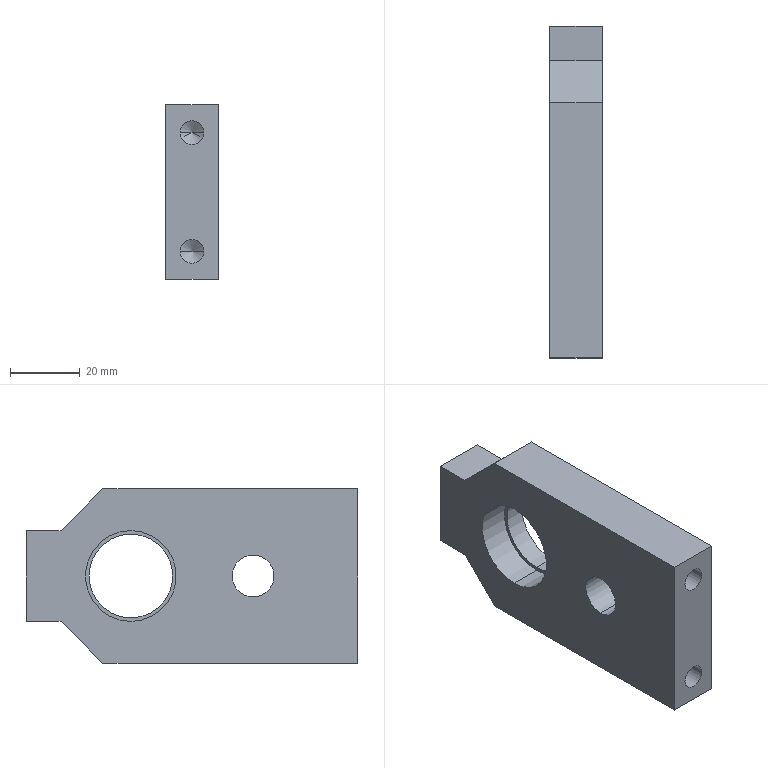Component | SolidWorks | BracketTwo-2 | 1 solid | 25 faces | box 15 x 95 x 50 mm | volume 55307 mm3 | plane 11 | cylinder 10 | cone 4 | commonest cylinder face diameters 6.8 x4 24 x2 26 x2 12 x2
build123d program:
from build123d import *

# Parameters (mm, degrees)
SKETCH1_R             = 6
BOSS_EXTRUDE1_DEPTH   = 15
SKETCH2_R             = 13
CUT_EXTRUDE1_DEPTH    = 9
SKETCH3_R             = 12
CUT_EXTRUDE2_DEPTH    = 6
M8_TAPPED_HOLE1_D     = 6.8
M8_TAPPED_HOLE1_DEPTH = 13
M8_TAPPED_HOLE1_TIP   = 2.043
SKETCH7_W             = 26
SKETCH7_H             = 15
BOSS_EXTRUDE2_DEPTH   = 10


with BuildPart() as part:
    # Sketch1 → Boss-Extrude1 (new body)
    with BuildSketch(Plane.XY):
        Polygon((-25, 30.5), (-13, 42.5), (13, 42.5), (25, 30.5), (25, -42.5), (-25, -42.5), align=None)
        with Locations((0, -12.5)):
            Circle(SKETCH1_R, mode=Mode.SUBTRACT)
    extrude(amount=BOSS_EXTRUDE1_DEPTH)

    # Sketch2 → Cut-Extrude1 (cut)
    with BuildSketch(Plane.XY.offset(15)):
        with Locations((0, 22.5)):
            Circle(SKETCH2_R)
    extrude(amount=-CUT_EXTRUDE1_DEPTH, mode=Mode.SUBTRACT)

    # Sketch3 → Cut-Extrude2 (cut)
    with BuildSketch(Plane.XY.offset(6)):
        with Locations((0, 22.5)):
            Circle(SKETCH3_R)
    extrude(amount=-CUT_EXTRUDE2_DEPTH, mode=Mode.SUBTRACT)

    # M8 Tapped Hole1
    with Locations(Plane(origin=(0, -42.5, 0), x_dir=(-1, 0, 0), z_dir=(0, -1, 0))):
        with Locations((17, -7.5), (-17, -7.5)):
            Hole(M8_TAPPED_HOLE1_D / 2, depth=M8_TAPPED_HOLE1_DEPTH)
            with Locations((0, 0, -(M8_TAPPED_HOLE1_DEPTH + M8_TAPPED_HOLE1_TIP / 2))):  # 118° drill point
                Cone(0, M8_TAPPED_HOLE1_D / 2, M8_TAPPED_HOLE1_TIP, mode=Mode.SUBTRACT)

    # Sketch7 → Boss-Extrude2 (add)
    with BuildSketch(Plane(origin=(0, 42.5, 0), x_dir=(1, 0, 0), z_dir=(0, 1, 0))):
        with Locations((0, -7.5)):
            Rectangle(SKETCH7_W, SKETCH7_H)
    extrude(amount=BOSS_EXTRUDE2_DEPTH)


solid = part.part

# Placed as in the assembly
solid = solid.moved(Location((195.546, 54.5, 438.671), (0, -90, 0)))
STEP:
#1=COLOUR_RGB('',0.7922,0.8196,0.9333);
#2=FILL_AREA_STYLE_COLOUR('',#1);
#3=FILL_AREA_STYLE('',(#2));
#4=SURFACE_STYLE_FILL_AREA(#3);
#5=SURFACE_SIDE_STYLE('',(#4));
#6=SURFACE_STYLE_USAGE(.BOTH.,#5);
#7=PRESENTATION_STYLE_ASSIGNMENT((#6));
#8=CARTESIAN_POINT('',(7.27,0.9843,16.601));
#9=VERTEX_POINT('',#8);
#10=CARTESIAN_POINT('',(7.537,0.9843,16.601));
#11=VERTEX_POINT('',#10);
#12=CARTESIAN_POINT('',(7.403,0.9843,16.601));
#13=DIRECTION('',(0.,-1.,0.));
#14=DIRECTION('',(1.,0.,-0.));
#15=AXIS2_PLACEMENT_3D('',#12,#13,#14);
#16=CIRCLE('',#15,0.1339);
#17=EDGE_CURVE('',#9,#11,#16,.T.);
#18=ORIENTED_EDGE('',*,*,#17,.F.);
#19=CARTESIAN_POINT('',(7.27,0.4724,16.601));
#20=VERTEX_POINT('',#19);
#21=CARTESIAN_POINT('',(7.27,0.4724,16.601));
#22=DIRECTION('',(0.,-1.,0.));
#23=VECTOR('',#22,39.37);
#24=LINE('',#21,#23);
#25=EDGE_CURVE('',#9,#20,#24,.T.);
#26=ORIENTED_EDGE('',*,*,#25,.T.);
#27=CARTESIAN_POINT('',(7.537,0.4724,16.601));
#28=VERTEX_POINT('',#27);
#29=CARTESIAN_POINT('',(7.403,0.4724,16.601));
#30=DIRECTION('',(0.,-1.,0.));
#31=DIRECTION('',(1.,0.,-0.));
#32=AXIS2_PLACEMENT_3D('',#29,#30,#31);
#33=CIRCLE('',#32,0.1339);
#34=EDGE_CURVE('',#20,#28,#33,.T.);
#35=ORIENTED_EDGE('',*,*,#34,.T.);
#36=CARTESIAN_POINT('',(7.537,0.4724,16.601));
#37=DIRECTION('',(0.,-1.,0.));
#38=VECTOR('',#37,39.37);
#39=LINE('',#36,#38);
#40=EDGE_CURVE('',#11,#28,#39,.T.);
#41=ORIENTED_EDGE('',*,*,#40,.F.);
#42=EDGE_LOOP('',(#18,#26,#35,#41));
#43=FACE_OUTER_BOUND('',#42,.T.);
#44=CARTESIAN_POINT('',(7.403,0.4724,16.601));
#45=DIRECTION('',(0.,-1.,0.));
#46=DIRECTION('',(1.,0.,-0.));
#47=AXIS2_PLACEMENT_3D('',#44,#45,#46);
#48=CYLINDRICAL_SURFACE('',#47,0.1339);
#49=ADVANCED_FACE('',(#43),#48,.F.);
#50=CARTESIAN_POINT('',(7.403,1.065,16.601));
#51=VERTEX_POINT('',#50);
#52=CARTESIAN_POINT('',(7.537,0.9843,16.601));
#53=DIRECTION('',(0.8572,-0.515,-0.));
#54=VECTOR('',#53,39.37);
#55=LINE('',#52,#54);
#56=EDGE_CURVE('',#51,#11,#55,.T.);
#57=ORIENTED_EDGE('',*,*,#56,.F.);
#58=CARTESIAN_POINT('',(7.27,0.9843,16.601));
#59=DIRECTION('',(-0.8572,-0.515,0.));
#60=VECTOR('',#59,39.37);
#61=LINE('',#58,#60);
#62=EDGE_CURVE('',#51,#9,#61,.T.);
#63=ORIENTED_EDGE('',*,*,#62,.T.);
#64=ORIENTED_EDGE('',*,*,#17,.T.);
#65=EDGE_LOOP('',(#57,#63,#64));
#66=FACE_OUTER_BOUND('',#65,.T.);
#67=CARTESIAN_POINT('',(7.403,0.9843,16.601));
#68=DIRECTION('',(0.,-1.,0.));
#69=DIRECTION('',(1.,0.,-0.));
#70=AXIS2_PLACEMENT_3D('',#67,#68,#69);
#71=CONICAL_SURFACE('',#70,0.1339,1.03);
#72=ADVANCED_FACE('',(#66),#71,.F.);
#73=CARTESIAN_POINT('',(7.27,0.9843,17.94));
#74=VERTEX_POINT('',#73);
#75=CARTESIAN_POINT('',(7.537,0.9843,17.94));
#76=VERTEX_POINT('',#75);
#77=CARTESIAN_POINT('',(7.403,0.9843,17.94));
#78=DIRECTION('',(0.,-1.,0.));
#79=DIRECTION('',(1.,0.,-0.));
#80=AXIS2_PLACEMENT_3D('',#77,#78,#79);
#81=CIRCLE('',#80,0.1339);
#82=EDGE_CURVE('',#74,#76,#81,.T.);
#83=ORIENTED_EDGE('',*,*,#82,.F.);
#84=CARTESIAN_POINT('',(7.27,0.4724,17.94));
#85=VERTEX_POINT('',#84);
#86=CARTESIAN_POINT('',(7.27,0.4724,17.94));
#87=DIRECTION('',(0.,-1.,0.));
#88=VECTOR('',#87,39.37);
#89=LINE('',#86,#88);
#90=EDGE_CURVE('',#74,#85,#89,.T.);
#91=ORIENTED_EDGE('',*,*,#90,.T.);
#92=CARTESIAN_POINT('',(7.537,0.4724,17.94));
#93=VERTEX_POINT('',#92);
#94=CARTESIAN_POINT('',(7.403,0.4724,17.94));
#95=DIRECTION('',(0.,-1.,0.));
#96=DIRECTION('',(1.,0.,-0.));
#97=AXIS2_PLACEMENT_3D('',#94,#95,#96);
#98=CIRCLE('',#97,0.1339);
#99=EDGE_CURVE('',#85,#93,#98,.T.);
#100=ORIENTED_EDGE('',*,*,#99,.T.);
#101=CARTESIAN_POINT('',(7.537,0.4724,17.94));
#102=DIRECTION('',(0.,-1.,0.));
#103=VECTOR('',#102,39.37);
#104=LINE('',#101,#103);
#105=EDGE_CURVE('',#76,#93,#104,.T.);
#106=ORIENTED_EDGE('',*,*,#105,.F.);
#107=EDGE_LOOP('',(#83,#91,#100,#106));
#108=FACE_OUTER_BOUND('',#107,.T.);
#109=CARTESIAN_POINT('',(7.403,0.4724,17.94));
#110=DIRECTION('',(0.,-1.,0.));
#111=DIRECTION('',(1.,0.,-0.));
#112=AXIS2_PLACEMENT_3D('',#109,#110,#111);
#113=CYLINDRICAL_SURFACE('',#112,0.1339);
#114=ADVANCED_FACE('',(#108),#113,.F.);
#115=CARTESIAN_POINT('',(7.403,1.065,17.94));
#116=VERTEX_POINT('',#115);
#117=CARTESIAN_POINT('',(7.537,0.9843,17.94));
#118=DIRECTION('',(0.8572,-0.515,-0.));
#119=VECTOR('',#118,39.37);
#120=LINE('',#117,#119);
#121=EDGE_CURVE('',#116,#76,#120,.T.);
#122=ORIENTED_EDGE('',*,*,#121,.F.);
#123=CARTESIAN_POINT('',(7.27,0.9843,17.94));
#124=DIRECTION('',(-0.8572,-0.515,0.));
#125=VECTOR('',#124,39.37);
#126=LINE('',#123,#125);
#127=EDGE_CURVE('',#116,#74,#126,.T.);
#128=ORIENTED_EDGE('',*,*,#127,.T.);
#129=ORIENTED_EDGE('',*,*,#82,.T.);
#130=EDGE_LOOP('',(#122,#128,#129));
#131=FACE_OUTER_BOUND('',#130,.T.);
#132=CARTESIAN_POINT('',(7.403,0.9843,17.94));
#133=DIRECTION('',(0.,-1.,0.));
#134=DIRECTION('',(1.,0.,-0.));
#135=AXIS2_PLACEMENT_3D('',#132,#133,#134);
#136=CONICAL_SURFACE('',#135,0.1339,1.03);
#137=ADVANCED_FACE('',(#131),#136,.F.);
#138=CARTESIAN_POINT('',(7.699,3.031,17.743));
#139=VERTEX_POINT('',#138);
#140=CARTESIAN_POINT('',(7.699,3.031,16.798));
#141=VERTEX_POINT('',#140);
#142=CARTESIAN_POINT('',(7.699,3.031,17.271));
#143=DIRECTION('',(1.,0.,-0.));
#144=DIRECTION('',(0.,0.,1.));
#145=AXIS2_PLACEMENT_3D('',#142,#143,#144);
#146=CIRCLE('',#145,0.4724);
#147=EDGE_CURVE('',#139,#141,#146,.T.);
#148=ORIENTED_EDGE('',*,*,#147,.T.);
#149=CARTESIAN_POINT('',(7.462,3.031,16.798));
#150=VERTEX_POINT('',#149);
#151=CARTESIAN_POINT('',(9.035,3.031,16.798));
#152=DIRECTION('',(-1.,-0.,0.));
#153=VECTOR('',#152,39.37);
#154=LINE('',#151,#153);
#155=EDGE_CURVE('',#141,#150,#154,.T.);
#156=ORIENTED_EDGE('',*,*,#155,.T.);
#157=CARTESIAN_POINT('',(7.462,3.031,17.743));
#158=VERTEX_POINT('',#157);
#159=CARTESIAN_POINT('',(7.462,3.031,17.271));
#160=DIRECTION('',(-1.,-0.,0.));
#161=DIRECTION('',(0.,0.,1.));
#162=AXIS2_PLACEMENT_3D('',#159,#160,#161);
#163=CIRCLE('',#162,0.4724);
#164=EDGE_CURVE('',#150,#158,#163,.T.);
#165=ORIENTED_EDGE('',*,*,#164,.T.);
#166=CARTESIAN_POINT('',(9.035,3.031,17.743));
#167=DIRECTION('',(-1.,-0.,0.));
#168=VECTOR('',#167,39.37);
#169=LINE('',#166,#168);
#170=EDGE_CURVE('',#139,#158,#169,.T.);
#171=ORIENTED_EDGE('',*,*,#170,.F.);
#172=EDGE_LOOP('',(#148,#156,#165,#171));
#173=FACE_OUTER_BOUND('',#172,.T.);
#174=CARTESIAN_POINT('',(9.035,3.031,17.271));
#175=DIRECTION('',(-1.,-0.,0.));
#176=DIRECTION('',(0.,0.,1.));
#177=AXIS2_PLACEMENT_3D('',#174,#175,#176);
#178=CYLINDRICAL_SURFACE('',#177,0.4724);
#179=ADVANCED_FACE('',(#173),#178,.F.);
#180=CARTESIAN_POINT('',(7.462,3.031,16.759));
#181=VERTEX_POINT('',#180);
#182=CARTESIAN_POINT('',(7.462,3.031,17.782));
#183=VERTEX_POINT('',#182);
#184=CARTESIAN_POINT('',(7.462,3.031,17.271));
#185=DIRECTION('',(-1.,-0.,0.));
#186=DIRECTION('',(0.,0.,1.));
#187=AXIS2_PLACEMENT_3D('',#184,#185,#186);
#188=CIRCLE('',#187,0.5118);
#189=EDGE_CURVE('',#181,#183,#188,.T.);
#190=ORIENTED_EDGE('',*,*,#189,.F.);
#191=CARTESIAN_POINT('',(7.108,3.031,16.759));
#192=VERTEX_POINT('',#191);
#193=CARTESIAN_POINT('',(7.462,3.031,16.759));
#194=DIRECTION('',(-1.,-0.,0.));
#195=VECTOR('',#194,39.37);
#196=LINE('',#193,#195);
#197=EDGE_CURVE('',#181,#192,#196,.T.);
#198=ORIENTED_EDGE('',*,*,#197,.T.);
#199=CARTESIAN_POINT('',(7.108,3.031,17.782));
#200=VERTEX_POINT('',#199);
#201=CARTESIAN_POINT('',(7.108,3.031,17.271));
#202=DIRECTION('',(-1.,-0.,0.));
#203=DIRECTION('',(0.,0.,1.));
#204=AXIS2_PLACEMENT_3D('',#201,#202,#203);
#205=CIRCLE('',#204,0.5118);
#206=EDGE_CURVE('',#192,#200,#205,.T.);
#207=ORIENTED_EDGE('',*,*,#206,.T.);
#208=CARTESIAN_POINT('',(7.462,3.031,17.782));
#209=DIRECTION('',(-1.,-0.,0.));
#210=VECTOR('',#209,39.37);
#211=LINE('',#208,#210);
#212=EDGE_CURVE('',#183,#200,#211,.T.);
#213=ORIENTED_EDGE('',*,*,#212,.F.);
#214=EDGE_LOOP('',(#190,#198,#207,#213));
#215=FACE_OUTER_BOUND('',#214,.T.);
#216=CARTESIAN_POINT('',(7.462,3.031,17.271));
#217=DIRECTION('',(-1.,-0.,0.));
#218=DIRECTION('',(0.,0.,1.));
#219=AXIS2_PLACEMENT_3D('',#216,#217,#218);
#220=CYLINDRICAL_SURFACE('',#219,0.5118);
#221=ADVANCED_FACE('',(#215),#220,.F.);
#222=CARTESIAN_POINT('',(7.108,1.654,17.034));
#223=VERTEX_POINT('',#222);
#224=CARTESIAN_POINT('',(7.108,1.654,17.507));
#225=VERTEX_POINT('',#224);
#226=CARTESIAN_POINT('',(7.108,1.654,17.271));
#227=DIRECTION('',(-1.,-0.,0.));
#228=DIRECTION('',(0.,0.,1.));
#229=AXIS2_PLACEMENT_3D('',#226,#227,#228);
#230=CIRCLE('',#229,0.2362);
#231=EDGE_CURVE('',#223,#225,#230,.T.);
#232=ORIENTED_EDGE('',*,*,#231,.T.);
#233=CARTESIAN_POINT('',(7.699,1.654,17.507));
#234=VERTEX_POINT('',#233);
#235=CARTESIAN_POINT('',(7.108,1.654,17.507));
#236=DIRECTION('',(1.,0.,-0.));
#237=VECTOR('',#236,39.37);
#238=LINE('',#235,#237);
#239=EDGE_CURVE('',#225,#234,#238,.T.);
#240=ORIENTED_EDGE('',*,*,#239,.T.);
#241=CARTESIAN_POINT('',(7.699,1.654,17.034));
#242=VERTEX_POINT('',#241);
#243=CARTESIAN_POINT('',(7.699,1.654,17.271));
#244=DIRECTION('',(-1.,-0.,0.));
#245=DIRECTION('',(0.,0.,1.));
#246=AXIS2_PLACEMENT_3D('',#243,#244,#245);
#247=CIRCLE('',#246,0.2362);
#248=EDGE_CURVE('',#242,#234,#247,.T.);
#249=ORIENTED_EDGE('',*,*,#248,.F.);
#250=CARTESIAN_POINT('',(7.108,1.654,17.034));
#251=DIRECTION('',(1.,0.,-0.));
#252=VECTOR('',#251,39.37);
#253=LINE('',#250,#252);
#254=EDGE_CURVE('',#223,#242,#253,.T.);
#255=ORIENTED_EDGE('',*,*,#254,.F.);
#256=EDGE_LOOP('',(#232,#240,#249,#255));
#257=FACE_OUTER_BOUND('',#256,.T.);
#258=CARTESIAN_POINT('',(7.108,1.654,17.271));
#259=DIRECTION('',(1.,0.,-0.));
#260=DIRECTION('',(-0.,0.,-1.));
#261=AXIS2_PLACEMENT_3D('',#258,#259,#260);
#262=CYLINDRICAL_SURFACE('',#261,0.2362);
#263=ADVANCED_FACE('',(#257),#262,.F.);
#264=CARTESIAN_POINT('',(7.108,3.031,17.271));
#265=DIRECTION('',(-1.,-0.,0.));
#266=DIRECTION('',(0.,0.,1.));
#267=AXIS2_PLACEMENT_3D('',#264,#265,#266);
#268=CIRCLE('',#267,0.5118);
#269=EDGE_CURVE('',#200,#192,#268,.T.);
#270=ORIENTED_EDGE('',*,*,#269,.F.);
#271=ORIENTED_EDGE('',*,*,#206,.F.);
#272=EDGE_LOOP('',(#270,#271));
#273=FACE_BOUND('',#272,.T.);
#274=CARTESIAN_POINT('',(7.108,0.4724,18.255));
#275=VERTEX_POINT('',#274);
#276=CARTESIAN_POINT('',(7.108,3.346,18.255));
#277=VERTEX_POINT('',#276);
#278=CARTESIAN_POINT('',(7.108,3.346,18.255));
#279=DIRECTION('',(-0.,1.,-0.));
#280=VECTOR('',#279,39.37);
#281=LINE('',#278,#280);
#282=EDGE_CURVE('',#275,#277,#281,.T.);
#283=ORIENTED_EDGE('',*,*,#282,.T.);
#284=CARTESIAN_POINT('',(7.108,3.819,17.782));
#285=VERTEX_POINT('',#284);
#286=CARTESIAN_POINT('',(7.108,3.819,17.782));
#287=DIRECTION('',(-0.,0.7071,-0.7071));
#288=VECTOR('',#287,39.37);
#289=LINE('',#286,#288);
#290=EDGE_CURVE('',#277,#285,#289,.T.);
#291=ORIENTED_EDGE('',*,*,#290,.T.);
#292=CARTESIAN_POINT('',(7.108,4.213,17.782));
#293=VERTEX_POINT('',#292);
#294=CARTESIAN_POINT('',(7.108,4.213,17.782));
#295=DIRECTION('',(0.,-1.,-0.));
#296=VECTOR('',#295,39.37);
#297=LINE('',#294,#296);
#298=EDGE_CURVE('',#293,#285,#297,.T.);
#299=ORIENTED_EDGE('',*,*,#298,.F.);
#300=CARTESIAN_POINT('',(7.108,4.213,16.759));
#301=VERTEX_POINT('',#300);
#302=CARTESIAN_POINT('',(7.108,4.213,16.759));
#303=DIRECTION('',(0.,-0.,1.));
#304=VECTOR('',#303,39.37);
#305=LINE('',#302,#304);
#306=EDGE_CURVE('',#301,#293,#305,.T.);
#307=ORIENTED_EDGE('',*,*,#306,.F.);
#308=CARTESIAN_POINT('',(7.108,3.819,16.759));
#309=VERTEX_POINT('',#308);
#310=CARTESIAN_POINT('',(7.108,4.213,16.759));
#311=DIRECTION('',(0.,-1.,-0.));
#312=VECTOR('',#311,39.37);
#313=LINE('',#310,#312);
#314=EDGE_CURVE('',#301,#309,#313,.T.);
#315=ORIENTED_EDGE('',*,*,#314,.T.);
#316=CARTESIAN_POINT('',(7.108,3.346,16.286));
#317=VERTEX_POINT('',#316);
#318=CARTESIAN_POINT('',(7.108,3.346,16.286));
#319=DIRECTION('',(-0.,-0.7071,-0.7071));
#320=VECTOR('',#319,39.37);
#321=LINE('',#318,#320);
#322=EDGE_CURVE('',#309,#317,#321,.T.);
#323=ORIENTED_EDGE('',*,*,#322,.T.);
#324=CARTESIAN_POINT('',(7.108,0.4724,16.286));
#325=VERTEX_POINT('',#324);
#326=CARTESIAN_POINT('',(7.108,3.346,16.286));
#327=DIRECTION('',(0.,-1.,0.));
#328=VECTOR('',#327,39.37);
#329=LINE('',#326,#328);
#330=EDGE_CURVE('',#317,#325,#329,.T.);
#331=ORIENTED_EDGE('',*,*,#330,.T.);
#332=CARTESIAN_POINT('',(7.108,0.4724,16.286));
#333=DIRECTION('',(0.,0.,1.));
#334=VECTOR('',#333,39.37);
#335=LINE('',#332,#334);
#336=EDGE_CURVE('',#325,#275,#335,.T.);
#337=ORIENTED_EDGE('',*,*,#336,.T.);
#338=EDGE_LOOP('',(#283,#291,#299,#307,#315,#323,#331,#337));
#339=FACE_OUTER_BOUND('',#338,.T.);
#340=ORIENTED_EDGE('',*,*,#231,.F.);
#341=CARTESIAN_POINT('',(7.108,1.654,17.271));
#342=DIRECTION('',(-1.,-0.,0.));
#343=DIRECTION('',(0.,0.,1.));
#344=AXIS2_PLACEMENT_3D('',#341,#342,#343);
#345=CIRCLE('',#344,0.2362);
#346=EDGE_CURVE('',#225,#223,#345,.T.);
#347=ORIENTED_EDGE('',*,*,#346,.F.);
#348=EDGE_LOOP('',(#340,#347));
#349=FACE_BOUND('',#348,.T.);
#350=CARTESIAN_POINT('',(7.108,2.146,17.271));
#351=DIRECTION('',(-1.,-0.,0.));
#352=DIRECTION('',(0.,0.,1.));
#353=AXIS2_PLACEMENT_3D('',#350,#351,#352);
#354=PLANE('',#353);
#355=ADVANCED_FACE('',(#273,#339,#349),#354,.T.);
#356=ORIENTED_EDGE('',*,*,#147,.F.);
#357=CARTESIAN_POINT('',(7.699,3.031,17.271));
#358=DIRECTION('',(1.,0.,-0.));
#359=DIRECTION('',(0.,0.,1.));
#360=AXIS2_PLACEMENT_3D('',#357,#358,#359);
#361=CIRCLE('',#360,0.4724);
#362=EDGE_CURVE('',#141,#139,#361,.T.);
#363=ORIENTED_EDGE('',*,*,#362,.F.);
#364=EDGE_LOOP('',(#356,#363));
#365=FACE_BOUND('',#364,.T.);
#366=CARTESIAN_POINT('',(7.699,0.4724,18.255));
#367=VERTEX_POINT('',#366);
#368=CARTESIAN_POINT('',(7.699,3.346,18.255));
#369=VERTEX_POINT('',#368);
#370=CARTESIAN_POINT('',(7.699,3.346,18.255));
#371=DIRECTION('',(-0.,1.,-0.));
#372=VECTOR('',#371,39.37);
#373=LINE('',#370,#372);
#374=EDGE_CURVE('',#367,#369,#373,.T.);
#375=ORIENTED_EDGE('',*,*,#374,.F.);
#376=CARTESIAN_POINT('',(7.699,0.4724,16.286));
#377=VERTEX_POINT('',#376);
#378=CARTESIAN_POINT('',(7.699,0.4724,16.286));
#379=DIRECTION('',(0.,0.,1.));
#380=VECTOR('',#379,39.37);
#381=LINE('',#378,#380);
#382=EDGE_CURVE('',#377,#367,#381,.T.);
#383=ORIENTED_EDGE('',*,*,#382,.F.);
#384=CARTESIAN_POINT('',(7.699,3.346,16.286));
#385=VERTEX_POINT('',#384);
#386=CARTESIAN_POINT('',(7.699,3.346,16.286));
#387=DIRECTION('',(0.,-1.,0.));
#388=VECTOR('',#387,39.37);
#389=LINE('',#386,#388);
#390=EDGE_CURVE('',#385,#377,#389,.T.);
#391=ORIENTED_EDGE('',*,*,#390,.F.);
#392=CARTESIAN_POINT('',(7.699,3.819,16.759));
#393=VERTEX_POINT('',#392);
#394=CARTESIAN_POINT('',(7.699,3.346,16.286));
#395=DIRECTION('',(-0.,-0.7071,-0.7071));
#396=VECTOR('',#395,39.37);
#397=LINE('',#394,#396);
#398=EDGE_CURVE('',#393,#385,#397,.T.);
#399=ORIENTED_EDGE('',*,*,#398,.F.);
#400=CARTESIAN_POINT('',(7.699,4.213,16.759));
#401=VERTEX_POINT('',#400);
#402=CARTESIAN_POINT('',(7.699,4.213,16.759));
#403=DIRECTION('',(0.,-1.,-0.));
#404=VECTOR('',#403,39.37);
#405=LINE('',#402,#404);
#406=EDGE_CURVE('',#401,#393,#405,.T.);
#407=ORIENTED_EDGE('',*,*,#406,.F.);
#408=CARTESIAN_POINT('',(7.699,4.213,17.782));
#409=VERTEX_POINT('',#408);
#410=CARTESIAN_POINT('',(7.699,4.213,16.759));
#411=DIRECTION('',(-0.,0.,-1.));
#412=VECTOR('',#411,39.37);
#413=LINE('',#410,#412);
#414=EDGE_CURVE('',#409,#401,#413,.T.);
#415=ORIENTED_EDGE('',*,*,#414,.F.);
#416=CARTESIAN_POINT('',(7.699,3.819,17.782));
#417=VERTEX_POINT('',#416);
#418=CARTESIAN_POINT('',(7.699,4.213,17.782));
#419=DIRECTION('',(0.,-1.,-0.));
#420=VECTOR('',#419,39.37);
#421=LINE('',#418,#420);
#422=EDGE_CURVE('',#409,#417,#421,.T.);
#423=ORIENTED_EDGE('',*,*,#422,.T.);
#424=CARTESIAN_POINT('',(7.699,3.819,17.782));
#425=DIRECTION('',(-0.,0.7071,-0.7071));
#426=VECTOR('',#425,39.37);
#427=LINE('',#424,#426);
#428=EDGE_CURVE('',#369,#417,#427,.T.);
#429=ORIENTED_EDGE('',*,*,#428,.F.);
#430=EDGE_LOOP('',(#375,#383,#391,#399,#407,#415,#423,#429));
#431=FACE_OUTER_BOUND('',#430,.T.);
#432=ORIENTED_EDGE('',*,*,#248,.T.);
#433=CARTESIAN_POINT('',(7.699,1.654,17.271));
#434=DIRECTION('',(-1.,-0.,0.));
#435=DIRECTION('',(0.,0.,1.));
#436=AXIS2_PLACEMENT_3D('',#433,#434,#435);
#437=CIRCLE('',#436,0.2362);
#438=EDGE_CURVE('',#234,#242,#437,.T.);
#439=ORIENTED_EDGE('',*,*,#438,.T.);
#440=EDGE_LOOP('',(#432,#439));
#441=FACE_BOUND('',#440,.T.);
#442=CARTESIAN_POINT('',(7.699,2.146,17.271));
#443=DIRECTION('',(-1.,-0.,0.));
#444=DIRECTION('',(0.,0.,1.));
#445=AXIS2_PLACEMENT_3D('',#442,#443,#444);
#446=PLANE('',#445);
#447=ADVANCED_FACE('',(#365,#431,#441),#446,.F.);
#448=ORIENTED_EDGE('',*,*,#374,.T.);
#449=CARTESIAN_POINT('',(7.108,3.346,18.255));
#450=DIRECTION('',(1.,0.,-0.));
#451=VECTOR('',#450,39.37);
#452=LINE('',#449,#451);
#453=EDGE_CURVE('',#277,#369,#452,.T.);
#454=ORIENTED_EDGE('',*,*,#453,.F.);
#455=ORIENTED_EDGE('',*,*,#282,.F.);
#456=CARTESIAN_POINT('',(7.108,0.4724,18.255));
#457=DIRECTION('',(1.,0.,-0.));
#458=VECTOR('',#457,39.37);
#459=LINE('',#456,#458);
#460=EDGE_CURVE('',#275,#367,#459,.T.);
#461=ORIENTED_EDGE('',*,*,#460,.T.);
#462=EDGE_LOOP('',(#448,#454,#455,#461));
#463=FACE_OUTER_BOUND('',#462,.T.);
#464=CARTESIAN_POINT('',(7.108,3.346,18.255));
#465=DIRECTION('',(-0.,-0.,-1.));
#466=DIRECTION('',(0.,-1.,0.));
#467=AXIS2_PLACEMENT_3D('',#464,#465,#466);
#468=PLANE('',#467);
#469=ADVANCED_FACE('',(#463),#468,.F.);
#470=ORIENTED_EDGE('',*,*,#428,.T.);
#471=CARTESIAN_POINT('',(7.108,3.819,17.782));
#472=DIRECTION('',(1.,0.,-0.));
#473=VECTOR('',#472,39.37);
#474=LINE('',#471,#473);
#475=EDGE_CURVE('',#285,#417,#474,.T.);
#476=ORIENTED_EDGE('',*,*,#475,.F.);
#477=ORIENTED_EDGE('',*,*,#290,.F.);
#478=ORIENTED_EDGE('',*,*,#453,.T.);
#479=EDGE_LOOP('',(#470,#476,#477,#478));
#480=FACE_OUTER_BOUND('',#479,.T.);
#481=CARTESIAN_POINT('',(7.108,3.819,17.782));
#482=DIRECTION('',(-0.,-0.7071,-0.7071));
#483=DIRECTION('',(0.,-0.7071,0.7071));
#484=AXIS2_PLACEMENT_3D('',#481,#482,#483);
#485=PLANE('',#484);
#486=ADVANCED_FACE('',(#480),#485,.F.);
#487=ORIENTED_EDGE('',*,*,#398,.T.);
#488=CARTESIAN_POINT('',(7.108,3.346,16.286));
#489=DIRECTION('',(1.,0.,-0.));
#490=VECTOR('',#489,39.37);
#491=LINE('',#488,#490);
#492=EDGE_CURVE('',#317,#385,#491,.T.);
#493=ORIENTED_EDGE('',*,*,#492,.F.);
#494=ORIENTED_EDGE('',*,*,#322,.F.);
#495=CARTESIAN_POINT('',(7.108,3.819,16.759));
#496=DIRECTION('',(1.,0.,-0.));
#497=VECTOR('',#496,39.37);
#498=LINE('',#495,#497);
#499=EDGE_CURVE('',#309,#393,#498,.T.);
#500=ORIENTED_EDGE('',*,*,#499,.T.);
#501=EDGE_LOOP('',(#487,#493,#494,#500));
#502=FACE_OUTER_BOUND('',#501,.T.);
#503=CARTESIAN_POINT('',(7.108,3.346,16.286));
#504=DIRECTION('',(0.,-0.7071,0.7071));
#505=DIRECTION('',(0.,0.7071,0.7071));
#506=AXIS2_PLACEMENT_3D('',#503,#504,#505);
#507=PLANE('',#506);
#508=ADVANCED_FACE('',(#502),#507,.F.);
#509=ORIENTED_EDGE('',*,*,#390,.T.);
#510=CARTESIAN_POINT('',(7.108,0.4724,16.286));
#511=DIRECTION('',(1.,0.,-0.));
#512=VECTOR('',#511,39.37);
#513=LINE('',#510,#512);
#514=EDGE_CURVE('',#325,#377,#513,.T.);
#515=ORIENTED_EDGE('',*,*,#514,.F.);
#516=ORIENTED_EDGE('',*,*,#330,.F.);
#517=ORIENTED_EDGE('',*,*,#492,.T.);
#518=EDGE_LOOP('',(#509,#515,#516,#517));
#519=FACE_OUTER_BOUND('',#518,.T.);
#520=CARTESIAN_POINT('',(7.108,3.346,16.286));
#521=DIRECTION('',(0.,0.,1.));
#522=DIRECTION('',(-0.,1.,-0.));
#523=AXIS2_PLACEMENT_3D('',#520,#521,#522);
#524=PLANE('',#523);
#525=ADVANCED_FACE('',(#519),#524,.F.);
#526=CARTESIAN_POINT('',(7.403,0.4724,16.601));
#527=DIRECTION('',(0.,-1.,0.));
#528=DIRECTION('',(1.,0.,-0.));
#529=AXIS2_PLACEMENT_3D('',#526,#527,#528);
#530=CIRCLE('',#529,0.1339);
#531=EDGE_CURVE('',#28,#20,#530,.T.);
#532=ORIENTED_EDGE('',*,*,#531,.F.);
#533=ORIENTED_EDGE('',*,*,#34,.F.);
#534=EDGE_LOOP('',(#532,#533));
#535=FACE_BOUND('',#534,.T.);
#536=CARTESIAN_POINT('',(7.403,0.4724,17.94));
#537=DIRECTION('',(0.,-1.,0.));
#538=DIRECTION('',(1.,0.,-0.));
#539=AXIS2_PLACEMENT_3D('',#536,#537,#538);
#540=CIRCLE('',#539,0.1339);
#541=EDGE_CURVE('',#93,#85,#540,.T.);
#542=ORIENTED_EDGE('',*,*,#541,.F.);
#543=ORIENTED_EDGE('',*,*,#99,.F.);
#544=EDGE_LOOP('',(#542,#543));
#545=FACE_BOUND('',#544,.T.);
#546=ORIENTED_EDGE('',*,*,#382,.T.);
#547=ORIENTED_EDGE('',*,*,#460,.F.);
#548=ORIENTED_EDGE('',*,*,#336,.F.);
#549=ORIENTED_EDGE('',*,*,#514,.T.);
#550=EDGE_LOOP('',(#546,#547,#548,#549));
#551=FACE_OUTER_BOUND('',#550,.T.);
#552=CARTESIAN_POINT('',(7.108,0.4724,16.286));
#553=DIRECTION('',(-0.,1.,-0.));
#554=DIRECTION('',(-1.,-0.,0.));
#555=AXIS2_PLACEMENT_3D('',#552,#553,#554);
#556=PLANE('',#555);
#557=ADVANCED_FACE('',(#535,#545,#551),#556,.F.);
#558=ORIENTED_EDGE('',*,*,#239,.F.);
#559=ORIENTED_EDGE('',*,*,#346,.T.);
#560=ORIENTED_EDGE('',*,*,#254,.T.);
#561=ORIENTED_EDGE('',*,*,#438,.F.);
#562=EDGE_LOOP('',(#558,#559,#560,#561));
#563=FACE_OUTER_BOUND('',#562,.T.);
#564=CARTESIAN_POINT('',(7.108,1.654,17.271));
#565=DIRECTION('',(1.,0.,-0.));
#566=DIRECTION('',(-0.,0.,-1.));
#567=AXIS2_PLACEMENT_3D('',#564,#565,#566);
#568=CYLINDRICAL_SURFACE('',#567,0.2362);
#569=ADVANCED_FACE('',(#563),#568,.F.);
#570=ORIENTED_EDGE('',*,*,#197,.F.);
#571=CARTESIAN_POINT('',(7.462,3.031,17.271));
#572=DIRECTION('',(-1.,-0.,0.));
#573=DIRECTION('',(0.,0.,1.));
#574=AXIS2_PLACEMENT_3D('',#571,#572,#573);
#575=CIRCLE('',#574,0.5118);
#576=EDGE_CURVE('',#183,#181,#575,.T.);
#577=ORIENTED_EDGE('',*,*,#576,.F.);
#578=ORIENTED_EDGE('',*,*,#212,.T.);
#579=ORIENTED_EDGE('',*,*,#269,.T.);
#580=EDGE_LOOP('',(#570,#577,#578,#579));
#581=FACE_OUTER_BOUND('',#580,.T.);
#582=CARTESIAN_POINT('',(7.462,3.031,17.271));
#583=DIRECTION('',(-1.,-0.,0.));
#584=DIRECTION('',(0.,0.,1.));
#585=AXIS2_PLACEMENT_3D('',#582,#583,#584);
#586=CYLINDRICAL_SURFACE('',#585,0.5118);
#587=ADVANCED_FACE('',(#581),#586,.F.);
#588=CARTESIAN_POINT('',(7.462,3.031,17.271));
#589=DIRECTION('',(-1.,-0.,0.));
#590=DIRECTION('',(0.,0.,1.));
#591=AXIS2_PLACEMENT_3D('',#588,#589,#590);
#592=CIRCLE('',#591,0.4724);
#593=EDGE_CURVE('',#158,#150,#592,.T.);
#594=ORIENTED_EDGE('',*,*,#593,.F.);
#595=ORIENTED_EDGE('',*,*,#164,.F.);
#596=EDGE_LOOP('',(#594,#595));
#597=FACE_BOUND('',#596,.T.);
#598=ORIENTED_EDGE('',*,*,#576,.T.);
#599=ORIENTED_EDGE('',*,*,#189,.T.);
#600=EDGE_LOOP('',(#598,#599));
#601=FACE_OUTER_BOUND('',#600,.T.);
#602=CARTESIAN_POINT('',(7.462,3.031,17.271));
#603=DIRECTION('',(-1.,-0.,0.));
#604=DIRECTION('',(0.,0.,1.));
#605=AXIS2_PLACEMENT_3D('',#602,#603,#604);
#606=PLANE('',#605);
#607=ADVANCED_FACE('',(#597,#601),#606,.T.);
#608=ORIENTED_EDGE('',*,*,#155,.F.);
#609=ORIENTED_EDGE('',*,*,#362,.T.);
#610=ORIENTED_EDGE('',*,*,#170,.T.);
#611=ORIENTED_EDGE('',*,*,#593,.T.);
#612=EDGE_LOOP('',(#608,#609,#610,#611));
#613=FACE_OUTER_BOUND('',#612,.T.);
#614=CARTESIAN_POINT('',(9.035,3.031,17.271));
#615=DIRECTION('',(-1.,-0.,0.));
#616=DIRECTION('',(0.,0.,1.));
#617=AXIS2_PLACEMENT_3D('',#614,#615,#616);
#618=CYLINDRICAL_SURFACE('',#617,0.4724);
#619=ADVANCED_FACE('',(#613),#618,.F.);
#620=ORIENTED_EDGE('',*,*,#127,.F.);
#621=ORIENTED_EDGE('',*,*,#121,.T.);
#622=CARTESIAN_POINT('',(7.403,0.9843,17.94));
#623=DIRECTION('',(0.,-1.,0.));
#624=DIRECTION('',(1.,0.,-0.));
#625=AXIS2_PLACEMENT_3D('',#622,#623,#624);
#626=CIRCLE('',#625,0.1339);
#627=EDGE_CURVE('',#76,#74,#626,.T.);
#628=ORIENTED_EDGE('',*,*,#627,.T.);
#629=EDGE_LOOP('',(#620,#621,#628));
#630=FACE_OUTER_BOUND('',#629,.T.);
#631=CARTESIAN_POINT('',(7.403,0.9843,17.94));
#632=DIRECTION('',(0.,-1.,0.));
#633=DIRECTION('',(1.,0.,-0.));
#634=AXIS2_PLACEMENT_3D('',#631,#632,#633);
#635=CONICAL_SURFACE('',#634,0.1339,1.03);
#636=ADVANCED_FACE('',(#630),#635,.F.);
#637=ORIENTED_EDGE('',*,*,#90,.F.);
#638=ORIENTED_EDGE('',*,*,#627,.F.);
#639=ORIENTED_EDGE('',*,*,#105,.T.);
#640=ORIENTED_EDGE('',*,*,#541,.T.);
#641=EDGE_LOOP('',(#637,#638,#639,#640));
#642=FACE_OUTER_BOUND('',#641,.T.);
#643=CARTESIAN_POINT('',(7.403,0.4724,17.94));
#644=DIRECTION('',(0.,-1.,0.));
#645=DIRECTION('',(1.,0.,-0.));
#646=AXIS2_PLACEMENT_3D('',#643,#644,#645);
#647=CYLINDRICAL_SURFACE('',#646,0.1339);
#648=ADVANCED_FACE('',(#642),#647,.F.);
#649=ORIENTED_EDGE('',*,*,#62,.F.);
#650=ORIENTED_EDGE('',*,*,#56,.T.);
#651=CARTESIAN_POINT('',(7.403,0.9843,16.601));
#652=DIRECTION('',(0.,-1.,0.));
#653=DIRECTION('',(1.,0.,-0.));
#654=AXIS2_PLACEMENT_3D('',#651,#652,#653);
#655=CIRCLE('',#654,0.1339);
#656=EDGE_CURVE('',#11,#9,#655,.T.);
#657=ORIENTED_EDGE('',*,*,#656,.T.);
#658=EDGE_LOOP('',(#649,#650,#657));
#659=FACE_OUTER_BOUND('',#658,.T.);
#660=CARTESIAN_POINT('',(7.403,0.9843,16.601));
#661=DIRECTION('',(0.,-1.,0.));
#662=DIRECTION('',(1.,0.,-0.));
#663=AXIS2_PLACEMENT_3D('',#660,#661,#662);
#664=CONICAL_SURFACE('',#663,0.1339,1.03);
#665=ADVANCED_FACE('',(#659),#664,.F.);
#666=ORIENTED_EDGE('',*,*,#25,.F.);
#667=ORIENTED_EDGE('',*,*,#656,.F.);
#668=ORIENTED_EDGE('',*,*,#40,.T.);
#669=ORIENTED_EDGE('',*,*,#531,.T.);
#670=EDGE_LOOP('',(#666,#667,#668,#669));
#671=FACE_OUTER_BOUND('',#670,.T.);
#672=CARTESIAN_POINT('',(7.403,0.4724,16.601));
#673=DIRECTION('',(0.,-1.,0.));
#674=DIRECTION('',(1.,0.,-0.));
#675=AXIS2_PLACEMENT_3D('',#672,#673,#674);
#676=CYLINDRICAL_SURFACE('',#675,0.1339);
#677=ADVANCED_FACE('',(#671),#676,.F.);
#678=ORIENTED_EDGE('',*,*,#499,.F.);
#679=ORIENTED_EDGE('',*,*,#314,.F.);
#680=CARTESIAN_POINT('',(7.699,4.213,16.759));
#681=DIRECTION('',(-1.,-0.,0.));
#682=VECTOR('',#681,39.37);
#683=LINE('',#680,#682);
#684=EDGE_CURVE('',#401,#301,#683,.T.);
#685=ORIENTED_EDGE('',*,*,#684,.F.);
#686=ORIENTED_EDGE('',*,*,#406,.T.);
#687=EDGE_LOOP('',(#678,#679,#685,#686));
#688=FACE_OUTER_BOUND('',#687,.T.);
#689=CARTESIAN_POINT('',(7.699,4.213,16.759));
#690=DIRECTION('',(0.,-0.,1.));
#691=DIRECTION('',(-0.,1.,0.));
#692=AXIS2_PLACEMENT_3D('',#689,#690,#691);
#693=PLANE('',#692);
#694=ADVANCED_FACE('',(#688),#693,.F.);
#695=ORIENTED_EDGE('',*,*,#475,.T.);
#696=ORIENTED_EDGE('',*,*,#422,.F.);
#697=CARTESIAN_POINT('',(7.699,4.213,17.782));
#698=DIRECTION('',(1.,0.,-0.));
#699=VECTOR('',#698,39.37);
#700=LINE('',#697,#699);
#701=EDGE_CURVE('',#293,#409,#700,.T.);
#702=ORIENTED_EDGE('',*,*,#701,.F.);
#703=ORIENTED_EDGE('',*,*,#298,.T.);
#704=EDGE_LOOP('',(#695,#696,#702,#703));
#705=FACE_OUTER_BOUND('',#704,.T.);
#706=CARTESIAN_POINT('',(7.699,4.213,17.782));
#707=DIRECTION('',(-0.,0.,-1.));
#708=DIRECTION('',(0.,-1.,-0.));
#709=AXIS2_PLACEMENT_3D('',#706,#707,#708);
#710=PLANE('',#709);
#711=ADVANCED_FACE('',(#705),#710,.F.);
#712=ORIENTED_EDGE('',*,*,#684,.T.);
#713=ORIENTED_EDGE('',*,*,#306,.T.);
#714=ORIENTED_EDGE('',*,*,#701,.T.);
#715=ORIENTED_EDGE('',*,*,#414,.T.);
#716=EDGE_LOOP('',(#712,#713,#714,#715));
#717=FACE_OUTER_BOUND('',#716,.T.);
#718=CARTESIAN_POINT('',(7.699,4.213,17.271));
#719=DIRECTION('',(-0.,1.,0.));
#720=DIRECTION('',(-0.,0.,-1.));
#721=AXIS2_PLACEMENT_3D('',#718,#719,#720);
#722=PLANE('',#721);
#723=ADVANCED_FACE('',(#717),#722,.T.);
#724=CLOSED_SHELL('',(#49,#72,#114,#137,#179,#221,#263,#355,#447,#469,#486,#508,#525,#557,#569,#587,#607,#619,#636,#648,#665,#677,#694,#711,#723));
#725=MANIFOLD_SOLID_BREP('',#724);
#726=STYLED_ITEM('',(#7),#725);
#727=PRESENTATION_LAYER_ASSIGNMENT('','',(#726));
#728=CARTESIAN_POINT('',(0.,0.,0.));
#729=DIRECTION('',(0.,0.,1.));
#730=DIRECTION('',(1.,0.,0.));
#731=AXIS2_PLACEMENT_3D('',#728,#729,#730);
#732=(LENGTH_UNIT()NAMED_UNIT(*)SI_UNIT($,.METRE.));
#733=LENGTH_MEASURE_WITH_UNIT(LENGTH_MEASURE(0.0254),#732);
#734=DIMENSIONAL_EXPONENTS(1.,0.,0.,0.,0.,0.,0.);
#735=(CONVERSION_BASED_UNIT('',#733)LENGTH_UNIT()NAMED_UNIT(#734));
#736=UNCERTAINTY_MEASURE_WITH_UNIT(LENGTH_MEASURE(0.00001),#735,'','');
#737=(NAMED_UNIT(*)PLANE_ANGLE_UNIT()SI_UNIT($,.RADIAN.));
#738=(NAMED_UNIT(*)SI_UNIT($,.STERADIAN.)SOLID_ANGLE_UNIT());
#739=(GEOMETRIC_REPRESENTATION_CONTEXT(3)GLOBAL_UNCERTAINTY_ASSIGNED_CONTEXT((#736))GLOBAL_UNIT_ASSIGNED_CONTEXT((#735,#737,#738))REPRESENTATION_CONTEXT('',''));
#740=ADVANCED_BREP_SHAPE_REPRESENTATION('',(#725,#731),#739);
#741=(LENGTH_UNIT()NAMED_UNIT(*)SI_UNIT($,.METRE.));
#742=LENGTH_MEASURE_WITH_UNIT(LENGTH_MEASURE(0.0254),#741);
#743=DIMENSIONAL_EXPONENTS(1.,0.,0.,0.,0.,0.,0.);
#744=(CONVERSION_BASED_UNIT('',#742)LENGTH_UNIT()NAMED_UNIT(#743));
#745=UNCERTAINTY_MEASURE_WITH_UNIT(LENGTH_MEASURE(0.00001),#744,'','');
#746=(NAMED_UNIT(*)PLANE_ANGLE_UNIT()SI_UNIT($,.RADIAN.));
#747=(NAMED_UNIT(*)SI_UNIT($,.STERADIAN.)SOLID_ANGLE_UNIT());
#748=(GEOMETRIC_REPRESENTATION_CONTEXT(3)GLOBAL_UNCERTAINTY_ASSIGNED_CONTEXT((#745))GLOBAL_UNIT_ASSIGNED_CONTEXT((#744,#746,#747))REPRESENTATION_CONTEXT('',''));
#749=MECHANICAL_DESIGN_GEOMETRIC_PRESENTATION_REPRESENTATION('',(#726),#748);